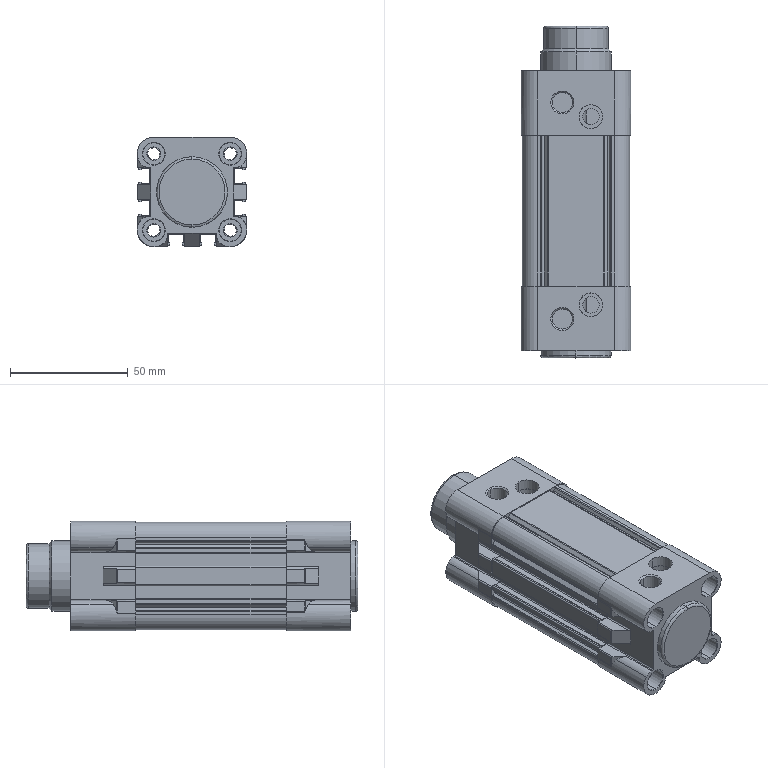Component | SolidWorks | HZ022-SE32x25S-1_HZ022-SE32x25S (2)-1 | 1 solid | 554 faces | volume 152541 mm3 | cylinder 276 | plane 248 | cone 26 | spline 4 | commonest cylinder face diameters 1 x104 0.4 x44 9.4 x16 5.8 x16 5.05 x12 8 x12 0.8 x12 14 x10 | material AL6061